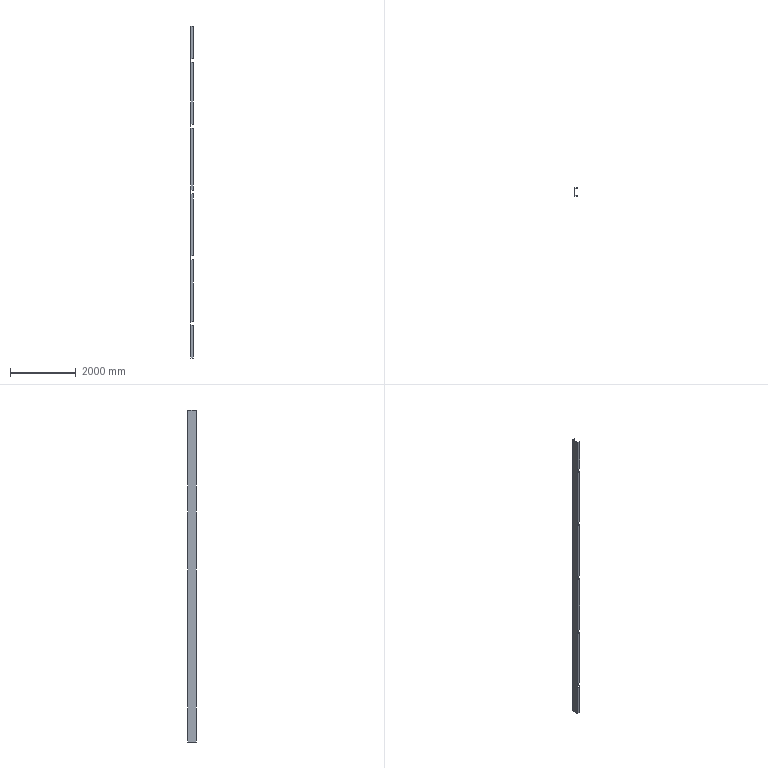Component | NX | CHUNSHUIJINCAO_5_1_2 | 1 solid | 50 faces | volume 38930040 mm3 | plane 50